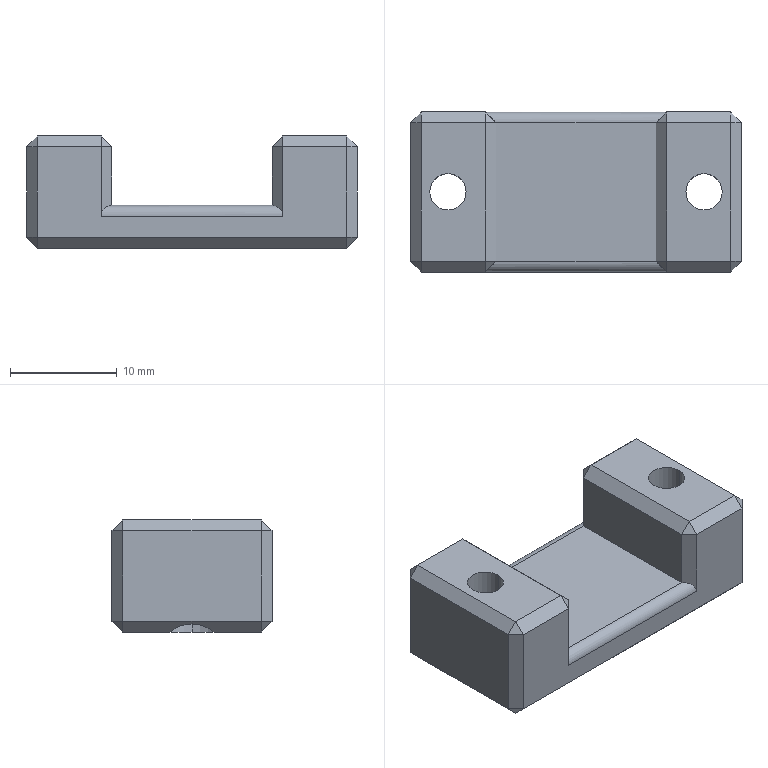CAM job | Mastercam | mm | 14 operations | part box 31 x 15 x 10.5
1. Contour (Ramp) | 9 - 10C 平底刀
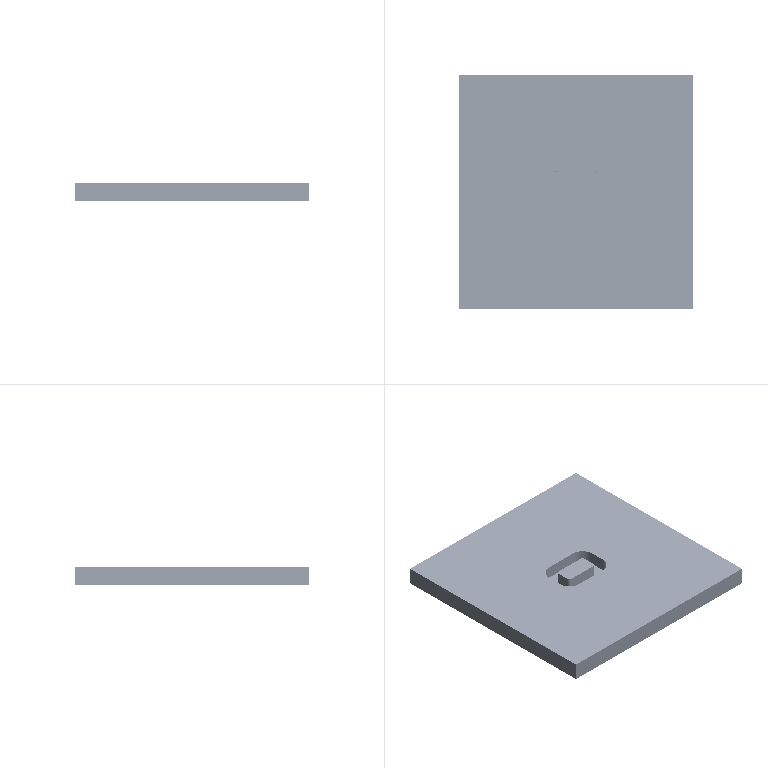2. 3D High Speed (Dynamic OptiRough) | 6 - 6 平底刀
3. Facing | 10 - 10J 平底刀
4. 3D High Speed (Waterline) | 20 - 4 -R0.5圆鼻铣刀
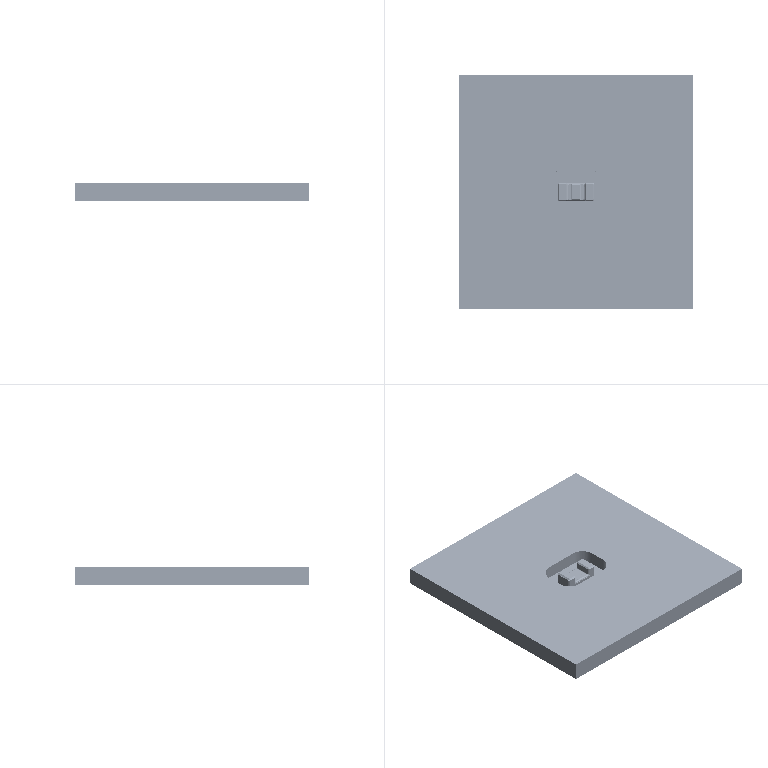5. Drill/Counterbore | 2 - 6定位倒角
6. Peck Drill | 12 - 3.4 钻头
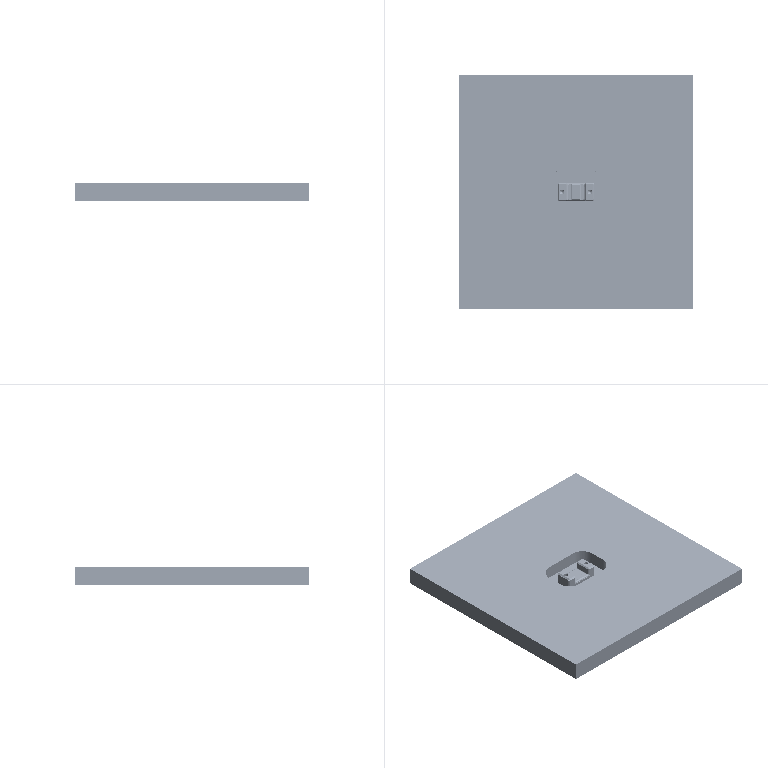7. 2D High Speed (2D Blend Mill) | 6 - 6 平底刀
8. Contour (2D chamfer) | 2 - 6定位倒角
9. Contour (Ramp) | 9 - 10C 平底刀
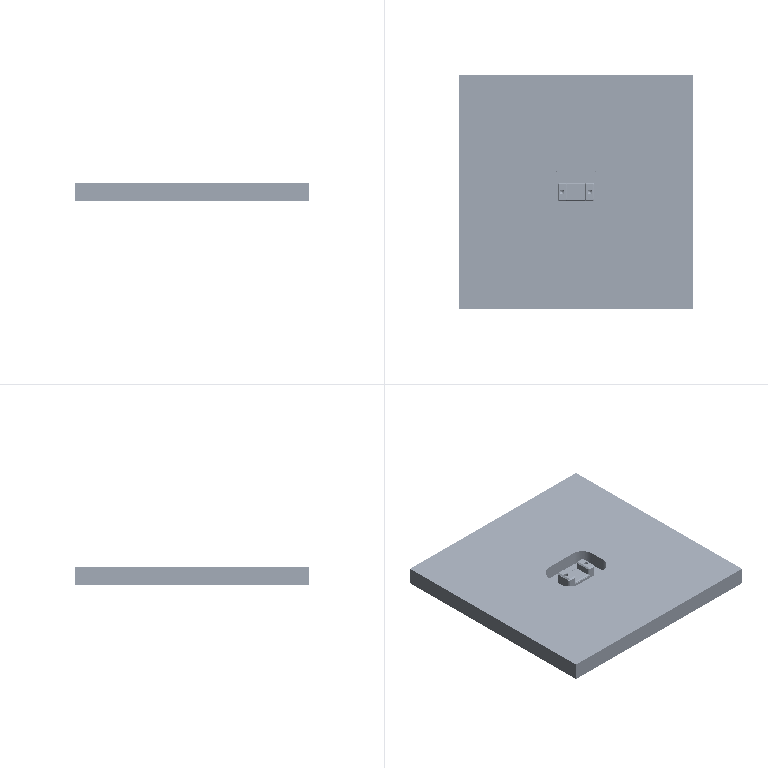10. Contour (2D) | 6 - 6 平底刀
11. Facing | 1 - 50 J面铣
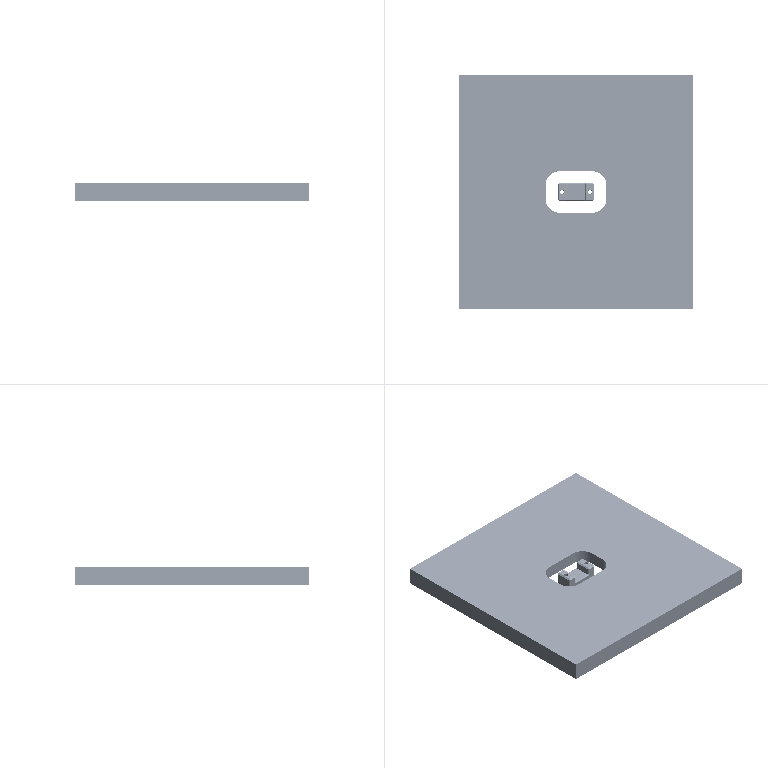12. Helix Bore | 7 - 4 平底刀
13. Contour (2D chamfer) | 2 - 6定位倒角
14. Unified Morph 5axis OP | 20 - 4 -R0.5圆鼻铣刀